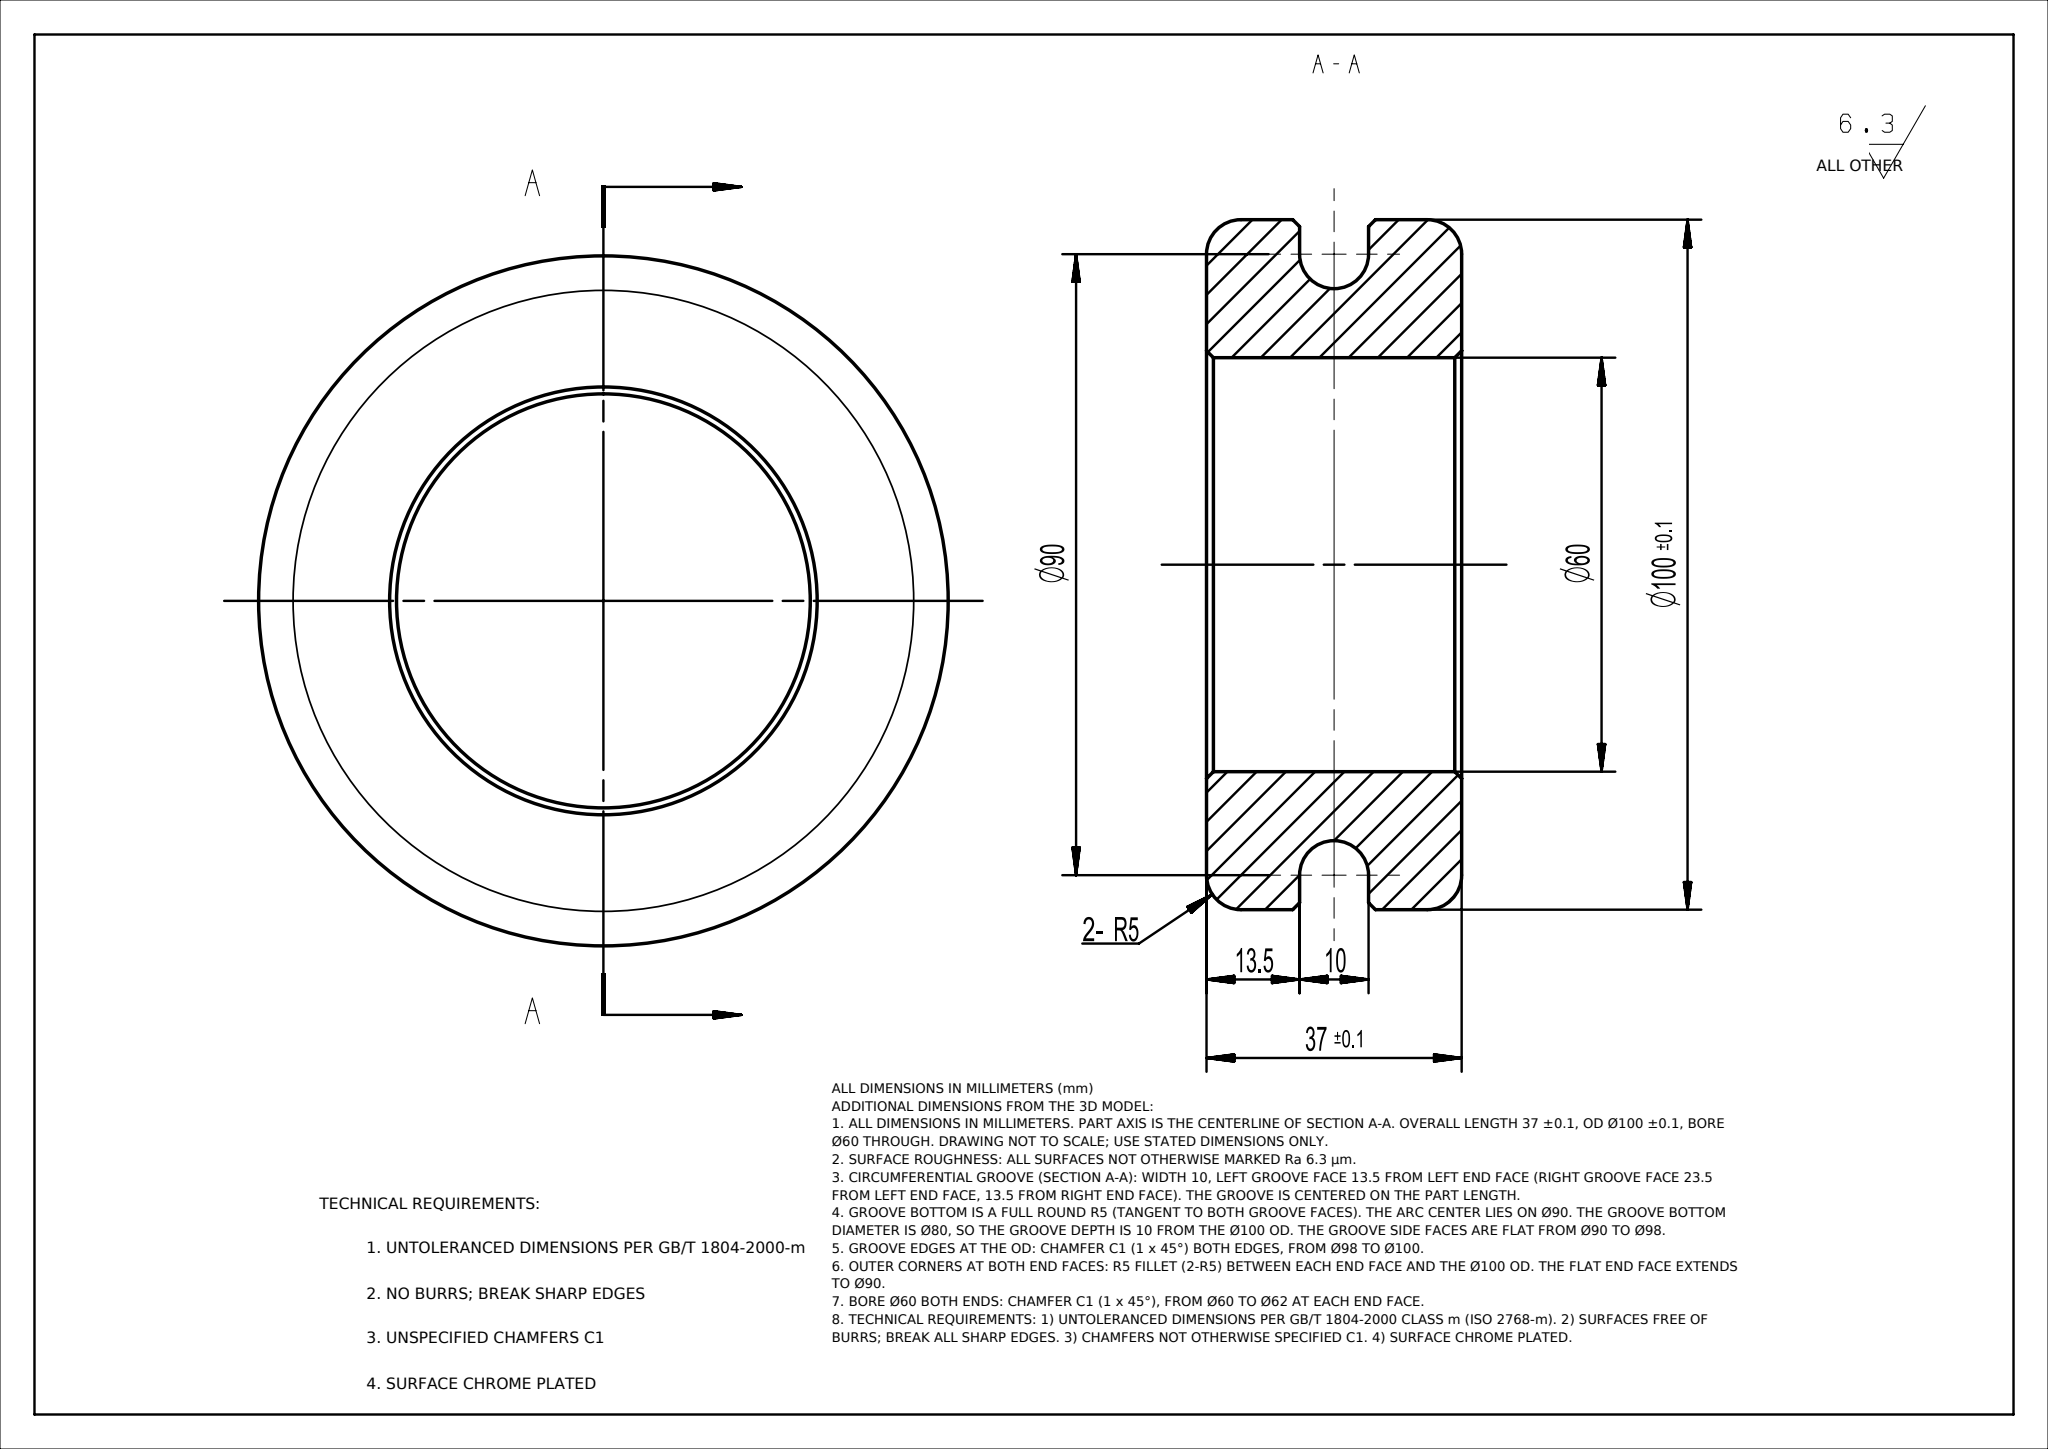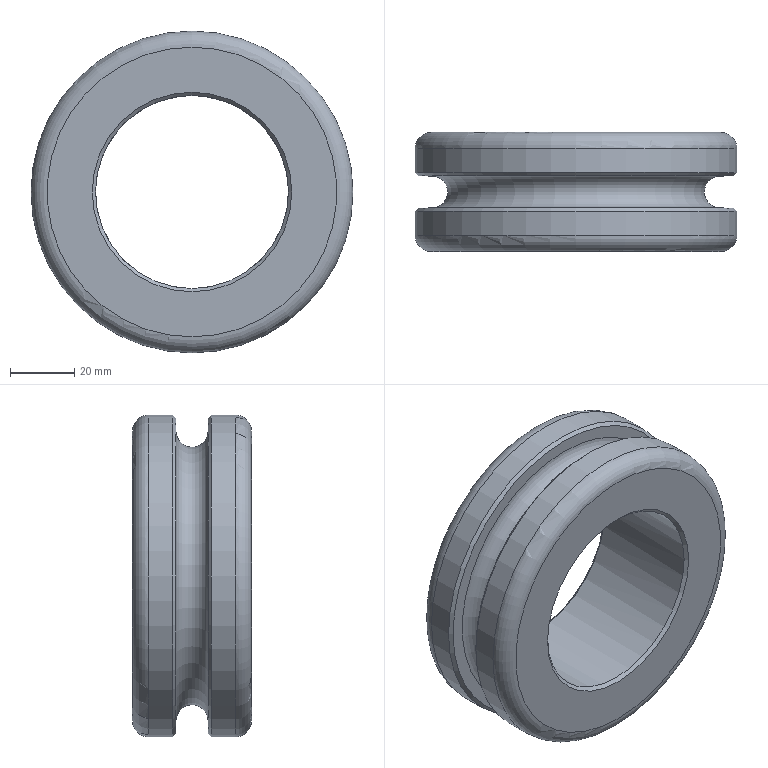Part | NX | mm | 1 solid | 14 faces | box 100 x 37 x 100 mm | volume 156682 mm3 | plane 4 | cone 4 | cylinder 3 | torus 3 | commonest cylinder face diameters 100 x2 60 x1
STEP:
#1=CARTESIAN_POINT('',(0.,0.,0.));
#2=DIRECTION('',(0.,0.,1.));
#3=DIRECTION('',(1.,0.,0.));
#4=AXIS2_PLACEMENT_3D('',#1,#2,#3);
#5=(LENGTH_UNIT()NAMED_UNIT(*)SI_UNIT(.MILLI.,.METRE.));
#6=UNCERTAINTY_MEASURE_WITH_UNIT(LENGTH_MEASURE(0.00002),#5,'','');
#7=(NAMED_UNIT(*)PLANE_ANGLE_UNIT()SI_UNIT($,.RADIAN.));
#8=PLANE_ANGLE_MEASURE_WITH_UNIT(PLANE_ANGLE_MEASURE(0.01745),#7);
#9=DIMENSIONAL_EXPONENTS(0.,0.,0.,0.,0.,0.,0.);
#10=(CONVERSION_BASED_UNIT('',#8)NAMED_UNIT(#9)PLANE_ANGLE_UNIT());
#11=(NAMED_UNIT(*)SI_UNIT($,.STERADIAN.)SOLID_ANGLE_UNIT());
#12=(GEOMETRIC_REPRESENTATION_CONTEXT(3)GLOBAL_UNCERTAINTY_ASSIGNED_CONTEXT((#6))GLOBAL_UNIT_ASSIGNED_CONTEXT((#5,#10,#11))REPRESENTATION_CONTEXT('',''));
#13=SHAPE_REPRESENTATION('',(#4),#12);
#14=CARTESIAN_POINT('',(0.,1.,45.));
#15=VERTEX_POINT('',#14);
#16=CARTESIAN_POINT('',(0.,1.,0.));
#17=DIRECTION('',(0.,-1.,0.));
#18=DIRECTION('',(0.,0.,1.));
#19=AXIS2_PLACEMENT_3D('',#16,#17,#18);
#20=CIRCLE('',#19,45.);
#21=EDGE_CURVE('',#15,#15,#20,.T.);
#22=ORIENTED_EDGE('',*,*,#21,.T.);
#23=EDGE_LOOP('',(#22));
#24=FACE_BOUND('',#23,.T.);
#25=CARTESIAN_POINT('',(0.,1.,31.));
#26=VERTEX_POINT('',#25);
#27=CARTESIAN_POINT('',(0.,1.,0.));
#28=DIRECTION('',(0.,1.,0.));
#29=DIRECTION('',(0.,0.,1.));
#30=AXIS2_PLACEMENT_3D('',#27,#28,#29);
#31=CIRCLE('',#30,31.);
#32=EDGE_CURVE('',#26,#26,#31,.T.);
#33=ORIENTED_EDGE('',*,*,#32,.T.);
#34=EDGE_LOOP('',(#33));
#35=FACE_BOUND('',#34,.T.);
#36=CARTESIAN_POINT('',(0.,1.,50.));
#37=DIRECTION('',(0.,1.,0.));
#38=DIRECTION('',(0.,0.,1.));
#39=AXIS2_PLACEMENT_3D('',#36,#37,#38);
#40=PLANE('',#39);
#41=ADVANCED_FACE('',(#24,#35),#40,.F.);
#42=CARTESIAN_POINT('',(0.,37.,-30.));
#43=VERTEX_POINT('',#42);
#44=CARTESIAN_POINT('',(0.,37.,0.));
#45=DIRECTION('',(0.,1.,0.));
#46=DIRECTION('',(0.,0.,-1.));
#47=AXIS2_PLACEMENT_3D('',#44,#45,#46);
#48=CIRCLE('',#47,30.);
#49=EDGE_CURVE('',#43,#43,#48,.T.);
#50=ORIENTED_EDGE('',*,*,#49,.T.);
#51=EDGE_LOOP('',(#50));
#52=FACE_BOUND('',#51,.T.);
#53=CARTESIAN_POINT('',(0.,2.,30.));
#54=VERTEX_POINT('',#53);
#55=CARTESIAN_POINT('',(0.,2.,0.));
#56=DIRECTION('',(0.,-1.,0.));
#57=DIRECTION('',(0.,0.,1.));
#58=AXIS2_PLACEMENT_3D('',#55,#56,#57);
#59=CIRCLE('',#58,30.);
#60=EDGE_CURVE('',#54,#54,#59,.T.);
#61=ORIENTED_EDGE('',*,*,#60,.T.);
#62=EDGE_LOOP('',(#61));
#63=FACE_BOUND('',#62,.T.);
#64=CARTESIAN_POINT('',(0.,0.,0.));
#65=DIRECTION('',(0.,-1.,0.));
#66=DIRECTION('',(0.,0.,-1.));
#67=AXIS2_PLACEMENT_3D('',#64,#65,#66);
#68=CYLINDRICAL_SURFACE('',#67,30.);
#69=ADVANCED_FACE('',(#52,#63),#68,.F.);
#70=CARTESIAN_POINT('',(0.,38.,-45.));
#71=VERTEX_POINT('',#70);
#72=CARTESIAN_POINT('',(0.,38.,0.));
#73=DIRECTION('',(0.,1.,0.));
#74=DIRECTION('',(0.,0.,-1.));
#75=AXIS2_PLACEMENT_3D('',#72,#73,#74);
#76=CIRCLE('',#75,45.);
#77=EDGE_CURVE('',#71,#71,#76,.T.);
#78=ORIENTED_EDGE('',*,*,#77,.T.);
#79=EDGE_LOOP('',(#78));
#80=FACE_BOUND('',#79,.T.);
#81=CARTESIAN_POINT('',(0.,38.,-31.));
#82=VERTEX_POINT('',#81);
#83=CARTESIAN_POINT('',(0.,38.,0.));
#84=DIRECTION('',(0.,-1.,0.));
#85=DIRECTION('',(0.,0.,-1.));
#86=AXIS2_PLACEMENT_3D('',#83,#84,#85);
#87=CIRCLE('',#86,31.);
#88=EDGE_CURVE('',#82,#82,#87,.T.);
#89=ORIENTED_EDGE('',*,*,#88,.T.);
#90=EDGE_LOOP('',(#89));
#91=FACE_BOUND('',#90,.T.);
#92=CARTESIAN_POINT('',(0.,38.,30.));
#93=DIRECTION('',(0.,-1.,0.));
#94=DIRECTION('',(0.,0.,-1.));
#95=AXIS2_PLACEMENT_3D('',#92,#93,#94);
#96=PLANE('',#95);
#97=ADVANCED_FACE('',(#80,#91),#96,.F.);
#98=CARTESIAN_POINT('',(0.,33.,-50.));
#99=VERTEX_POINT('',#98);
#100=CARTESIAN_POINT('',(0.,33.,0.));
#101=DIRECTION('',(0.,-1.,0.));
#102=DIRECTION('',(0.,0.,-1.));
#103=AXIS2_PLACEMENT_3D('',#100,#101,#102);
#104=CIRCLE('',#103,50.);
#105=EDGE_CURVE('',#99,#99,#104,.T.);
#106=ORIENTED_EDGE('',*,*,#105,.T.);
#107=EDGE_LOOP('',(#106));
#108=FACE_BOUND('',#107,.T.);
#109=CARTESIAN_POINT('',(0.,25.5,50.));
#110=VERTEX_POINT('',#109);
#111=CARTESIAN_POINT('',(0.,25.5,0.));
#112=DIRECTION('',(0.,1.,0.));
#113=DIRECTION('',(0.,0.,1.));
#114=AXIS2_PLACEMENT_3D('',#111,#112,#113);
#115=CIRCLE('',#114,50.);
#116=EDGE_CURVE('',#110,#110,#115,.T.);
#117=ORIENTED_EDGE('',*,*,#116,.T.);
#118=EDGE_LOOP('',(#117));
#119=FACE_BOUND('',#118,.T.);
#120=CARTESIAN_POINT('',(0.,0.,0.));
#121=DIRECTION('',(0.,-1.,0.));
#122=DIRECTION('',(0.,0.,-1.));
#123=AXIS2_PLACEMENT_3D('',#120,#121,#122);
#124=CYLINDRICAL_SURFACE('',#123,50.);
#125=ADVANCED_FACE('',(#108,#119),#124,.T.);
#126=CARTESIAN_POINT('',(0.,24.5,49.));
#127=VERTEX_POINT('',#126);
#128=CARTESIAN_POINT('',(0.,24.5,0.));
#129=DIRECTION('',(0.,-1.,0.));
#130=DIRECTION('',(0.,0.,1.));
#131=AXIS2_PLACEMENT_3D('',#128,#129,#130);
#132=CIRCLE('',#131,49.);
#133=EDGE_CURVE('',#127,#127,#132,.T.);
#134=ORIENTED_EDGE('',*,*,#133,.T.);
#135=EDGE_LOOP('',(#134));
#136=FACE_BOUND('',#135,.T.);
#137=CARTESIAN_POINT('',(0.,24.5,-45.));
#138=VERTEX_POINT('',#137);
#139=CARTESIAN_POINT('',(0.,24.5,0.));
#140=DIRECTION('',(0.,-1.,0.));
#141=DIRECTION('',(0.,0.,-1.));
#142=AXIS2_PLACEMENT_3D('',#139,#140,#141);
#143=CIRCLE('',#142,45.);
#144=EDGE_CURVE('',#138,#138,#143,.T.);
#145=ORIENTED_EDGE('',*,*,#144,.F.);
#146=EDGE_LOOP('',(#145));
#147=FACE_BOUND('',#146,.T.);
#148=CARTESIAN_POINT('',(0.,24.5,50.));
#149=DIRECTION('',(0.,1.,0.));
#150=DIRECTION('',(0.,0.,1.));
#151=AXIS2_PLACEMENT_3D('',#148,#149,#150);
#152=PLANE('',#151);
#153=ADVANCED_FACE('',(#136,#147),#152,.F.);
#154=CARTESIAN_POINT('',(0.,14.5,-45.));
#155=VERTEX_POINT('',#154);
#156=CARTESIAN_POINT('',(0.,14.5,0.));
#157=DIRECTION('',(0.,-1.,0.));
#158=DIRECTION('',(0.,0.,-1.));
#159=AXIS2_PLACEMENT_3D('',#156,#157,#158);
#160=CIRCLE('',#159,45.);
#161=EDGE_CURVE('',#155,#155,#160,.T.);
#162=ORIENTED_EDGE('',*,*,#161,.F.);
#163=EDGE_LOOP('',(#162));
#164=FACE_BOUND('',#163,.T.);
#165=ORIENTED_EDGE('',*,*,#144,.T.);
#166=EDGE_LOOP('',(#165));
#167=FACE_BOUND('',#166,.T.);
#168=CARTESIAN_POINT('',(0.,19.5,0.));
#169=DIRECTION('',(0.,-1.,0.));
#170=DIRECTION('',(0.,0.,-1.));
#171=AXIS2_PLACEMENT_3D('',#168,#169,#170);
#172=TOROIDAL_SURFACE('',#171,45.,5.);
#173=ADVANCED_FACE('',(#164,#167),#172,.F.);
#174=CARTESIAN_POINT('',(0.,14.5,-49.));
#175=VERTEX_POINT('',#174);
#176=CARTESIAN_POINT('',(0.,14.5,0.));
#177=DIRECTION('',(0.,1.,0.));
#178=DIRECTION('',(0.,0.,-1.));
#179=AXIS2_PLACEMENT_3D('',#176,#177,#178);
#180=CIRCLE('',#179,49.);
#181=EDGE_CURVE('',#175,#175,#180,.T.);
#182=ORIENTED_EDGE('',*,*,#181,.T.);
#183=EDGE_LOOP('',(#182));
#184=FACE_BOUND('',#183,.T.);
#185=ORIENTED_EDGE('',*,*,#161,.T.);
#186=EDGE_LOOP('',(#185));
#187=FACE_BOUND('',#186,.T.);
#188=CARTESIAN_POINT('',(0.,14.5,45.));
#189=DIRECTION('',(0.,-1.,0.));
#190=DIRECTION('',(0.,0.,-1.));
#191=AXIS2_PLACEMENT_3D('',#188,#189,#190);
#192=PLANE('',#191);
#193=ADVANCED_FACE('',(#184,#187),#192,.F.);
#194=CARTESIAN_POINT('',(0.,6.,50.));
#195=VERTEX_POINT('',#194);
#196=CARTESIAN_POINT('',(0.,6.,0.));
#197=DIRECTION('',(0.,1.,0.));
#198=DIRECTION('',(0.,0.,1.));
#199=AXIS2_PLACEMENT_3D('',#196,#197,#198);
#200=CIRCLE('',#199,50.);
#201=EDGE_CURVE('',#195,#195,#200,.T.);
#202=ORIENTED_EDGE('',*,*,#201,.T.);
#203=EDGE_LOOP('',(#202));
#204=FACE_BOUND('',#203,.T.);
#205=CARTESIAN_POINT('',(0.,13.5,-50.));
#206=VERTEX_POINT('',#205);
#207=CARTESIAN_POINT('',(0.,13.5,0.));
#208=DIRECTION('',(0.,-1.,0.));
#209=DIRECTION('',(0.,0.,-1.));
#210=AXIS2_PLACEMENT_3D('',#207,#208,#209);
#211=CIRCLE('',#210,50.);
#212=EDGE_CURVE('',#206,#206,#211,.T.);
#213=ORIENTED_EDGE('',*,*,#212,.T.);
#214=EDGE_LOOP('',(#213));
#215=FACE_BOUND('',#214,.T.);
#216=CARTESIAN_POINT('',(0.,0.,0.));
#217=DIRECTION('',(0.,-1.,0.));
#218=DIRECTION('',(0.,0.,-1.));
#219=AXIS2_PLACEMENT_3D('',#216,#217,#218);
#220=CYLINDRICAL_SURFACE('',#219,50.);
#221=ADVANCED_FACE('',(#204,#215),#220,.T.);
#222=ORIENTED_EDGE('',*,*,#49,.F.);
#223=EDGE_LOOP('',(#222));
#224=FACE_BOUND('',#223,.T.);
#225=ORIENTED_EDGE('',*,*,#88,.F.);
#226=EDGE_LOOP('',(#225));
#227=FACE_BOUND('',#226,.T.);
#228=CARTESIAN_POINT('',(0.,38.,0.));
#229=DIRECTION('',(0.,1.,0.));
#230=DIRECTION('',(0.,0.,1.));
#231=AXIS2_PLACEMENT_3D('',#228,#229,#230);
#232=CONICAL_SURFACE('',#231,31.,45.);
#233=ADVANCED_FACE('',(#224,#227),#232,.F.);
#234=ORIENTED_EDGE('',*,*,#32,.F.);
#235=EDGE_LOOP('',(#234));
#236=FACE_BOUND('',#235,.T.);
#237=ORIENTED_EDGE('',*,*,#60,.F.);
#238=EDGE_LOOP('',(#237));
#239=FACE_BOUND('',#238,.T.);
#240=CARTESIAN_POINT('',(0.,2.,0.));
#241=DIRECTION('',(0.,-1.,0.));
#242=DIRECTION('',(0.,0.,-1.));
#243=AXIS2_PLACEMENT_3D('',#240,#241,#242);
#244=CONICAL_SURFACE('',#243,30.,45.);
#245=ADVANCED_FACE('',(#236,#239),#244,.F.);
#246=ORIENTED_EDGE('',*,*,#181,.F.);
#247=EDGE_LOOP('',(#246));
#248=FACE_BOUND('',#247,.T.);
#249=ORIENTED_EDGE('',*,*,#212,.F.);
#250=EDGE_LOOP('',(#249));
#251=FACE_BOUND('',#250,.T.);
#252=CARTESIAN_POINT('',(0.,13.5,0.));
#253=DIRECTION('',(0.,-1.,0.));
#254=DIRECTION('',(0.,-0.,-1.));
#255=AXIS2_PLACEMENT_3D('',#252,#253,#254);
#256=CONICAL_SURFACE('',#255,50.,45.);
#257=ADVANCED_FACE('',(#248,#251),#256,.T.);
#258=ORIENTED_EDGE('',*,*,#116,.F.);
#259=EDGE_LOOP('',(#258));
#260=FACE_BOUND('',#259,.T.);
#261=ORIENTED_EDGE('',*,*,#133,.F.);
#262=EDGE_LOOP('',(#261));
#263=FACE_BOUND('',#262,.T.);
#264=CARTESIAN_POINT('',(0.,24.5,0.));
#265=DIRECTION('',(0.,1.,0.));
#266=DIRECTION('',(0.,-0.,1.));
#267=AXIS2_PLACEMENT_3D('',#264,#265,#266);
#268=CONICAL_SURFACE('',#267,49.,45.);
#269=ADVANCED_FACE('',(#260,#263),#268,.T.);
#270=ORIENTED_EDGE('',*,*,#201,.F.);
#271=EDGE_LOOP('',(#270));
#272=FACE_BOUND('',#271,.T.);
#273=ORIENTED_EDGE('',*,*,#21,.F.);
#274=EDGE_LOOP('',(#273));
#275=FACE_BOUND('',#274,.T.);
#276=CARTESIAN_POINT('',(0.,6.,0.));
#277=DIRECTION('',(0.,1.,0.));
#278=DIRECTION('',(0.,0.,1.));
#279=AXIS2_PLACEMENT_3D('',#276,#277,#278);
#280=TOROIDAL_SURFACE('',#279,45.,5.);
#281=ADVANCED_FACE('',(#272,#275),#280,.T.);
#282=ORIENTED_EDGE('',*,*,#77,.F.);
#283=EDGE_LOOP('',(#282));
#284=FACE_BOUND('',#283,.T.);
#285=ORIENTED_EDGE('',*,*,#105,.F.);
#286=EDGE_LOOP('',(#285));
#287=FACE_BOUND('',#286,.T.);
#288=CARTESIAN_POINT('',(0.,33.,0.));
#289=DIRECTION('',(0.,-1.,0.));
#290=DIRECTION('',(0.,0.,-1.));
#291=AXIS2_PLACEMENT_3D('',#288,#289,#290);
#292=TOROIDAL_SURFACE('',#291,45.,5.);
#293=ADVANCED_FACE('',(#284,#287),#292,.T.);
#294=CLOSED_SHELL('',(#41,#69,#97,#125,#153,#173,#193,#221,#233,#245,#257,#269,#281,#293));
#295=MANIFOLD_SOLID_BREP('',#294);
#296=ADVANCED_BREP_SHAPE_REPRESENTATION('',(#295),#12);
#297=SHAPE_REPRESENTATION_RELATIONSHIP('','',#13,#296);
#298=PRESENTATION_LAYER_ASSIGNMENT('','',(#295));
#299=COLOUR_RGB('',0.8,0.8,0.8);
#300=FILL_AREA_STYLE_COLOUR('',#299);
#301=FILL_AREA_STYLE('',(#300));
#302=SURFACE_STYLE_FILL_AREA(#301);
#303=SURFACE_SIDE_STYLE('',(#302));
#304=SURFACE_STYLE_USAGE(.BOTH.,#303);
#305=PRESENTATION_STYLE_ASSIGNMENT((#304));
#306=STYLED_ITEM('',(#305),#295);
#307=MECHANICAL_DESIGN_GEOMETRIC_PRESENTATION_REPRESENTATION('',(#306),#12);